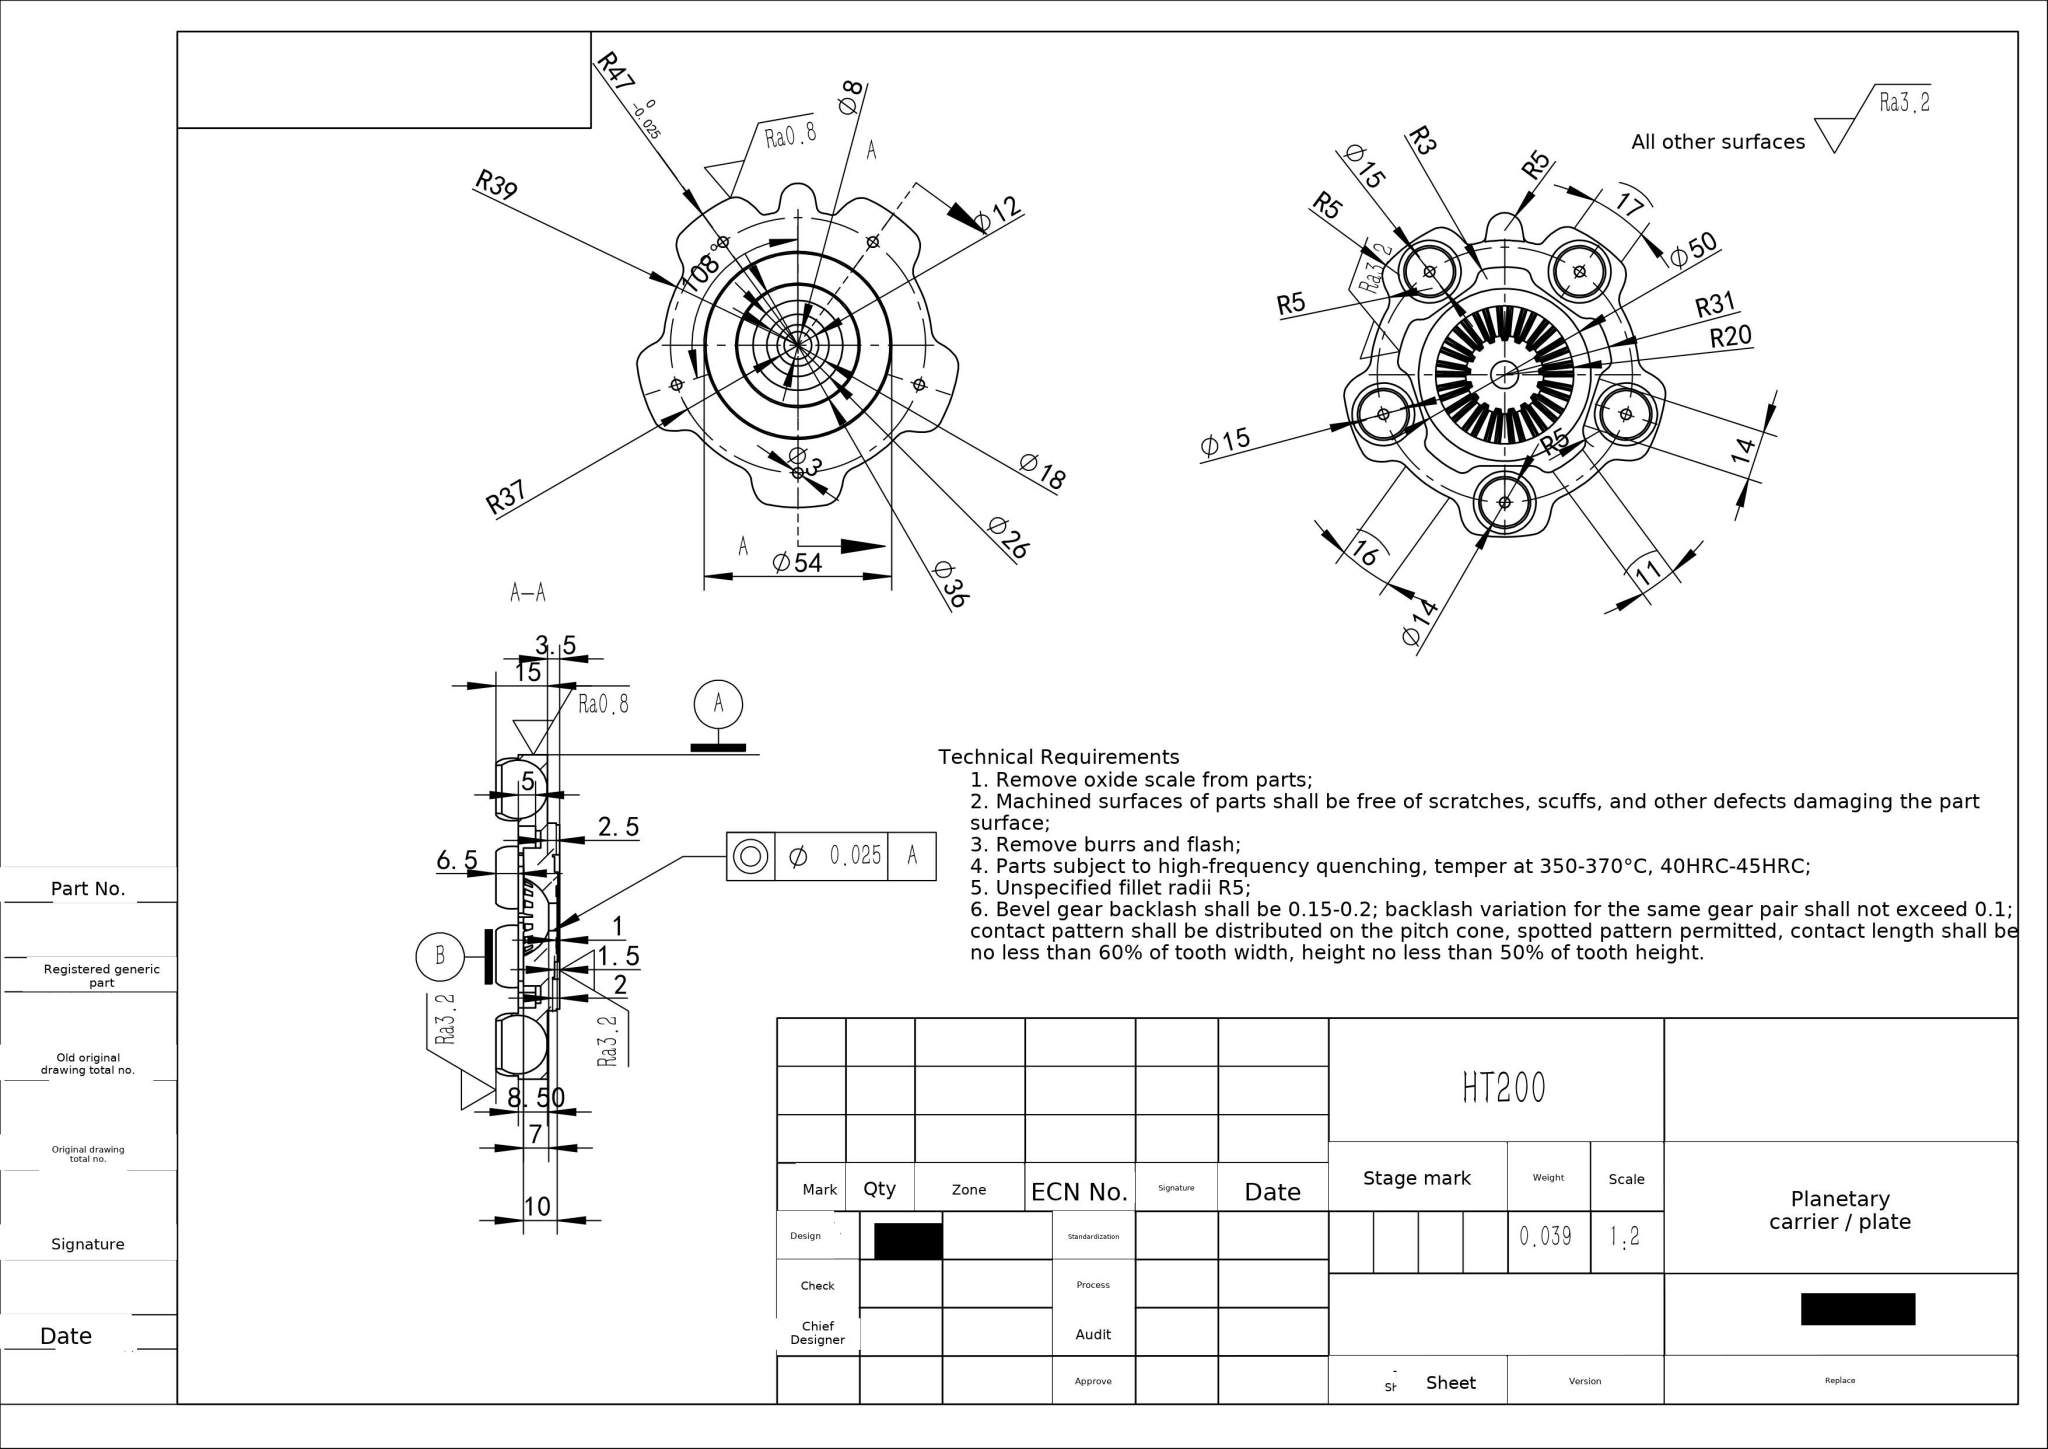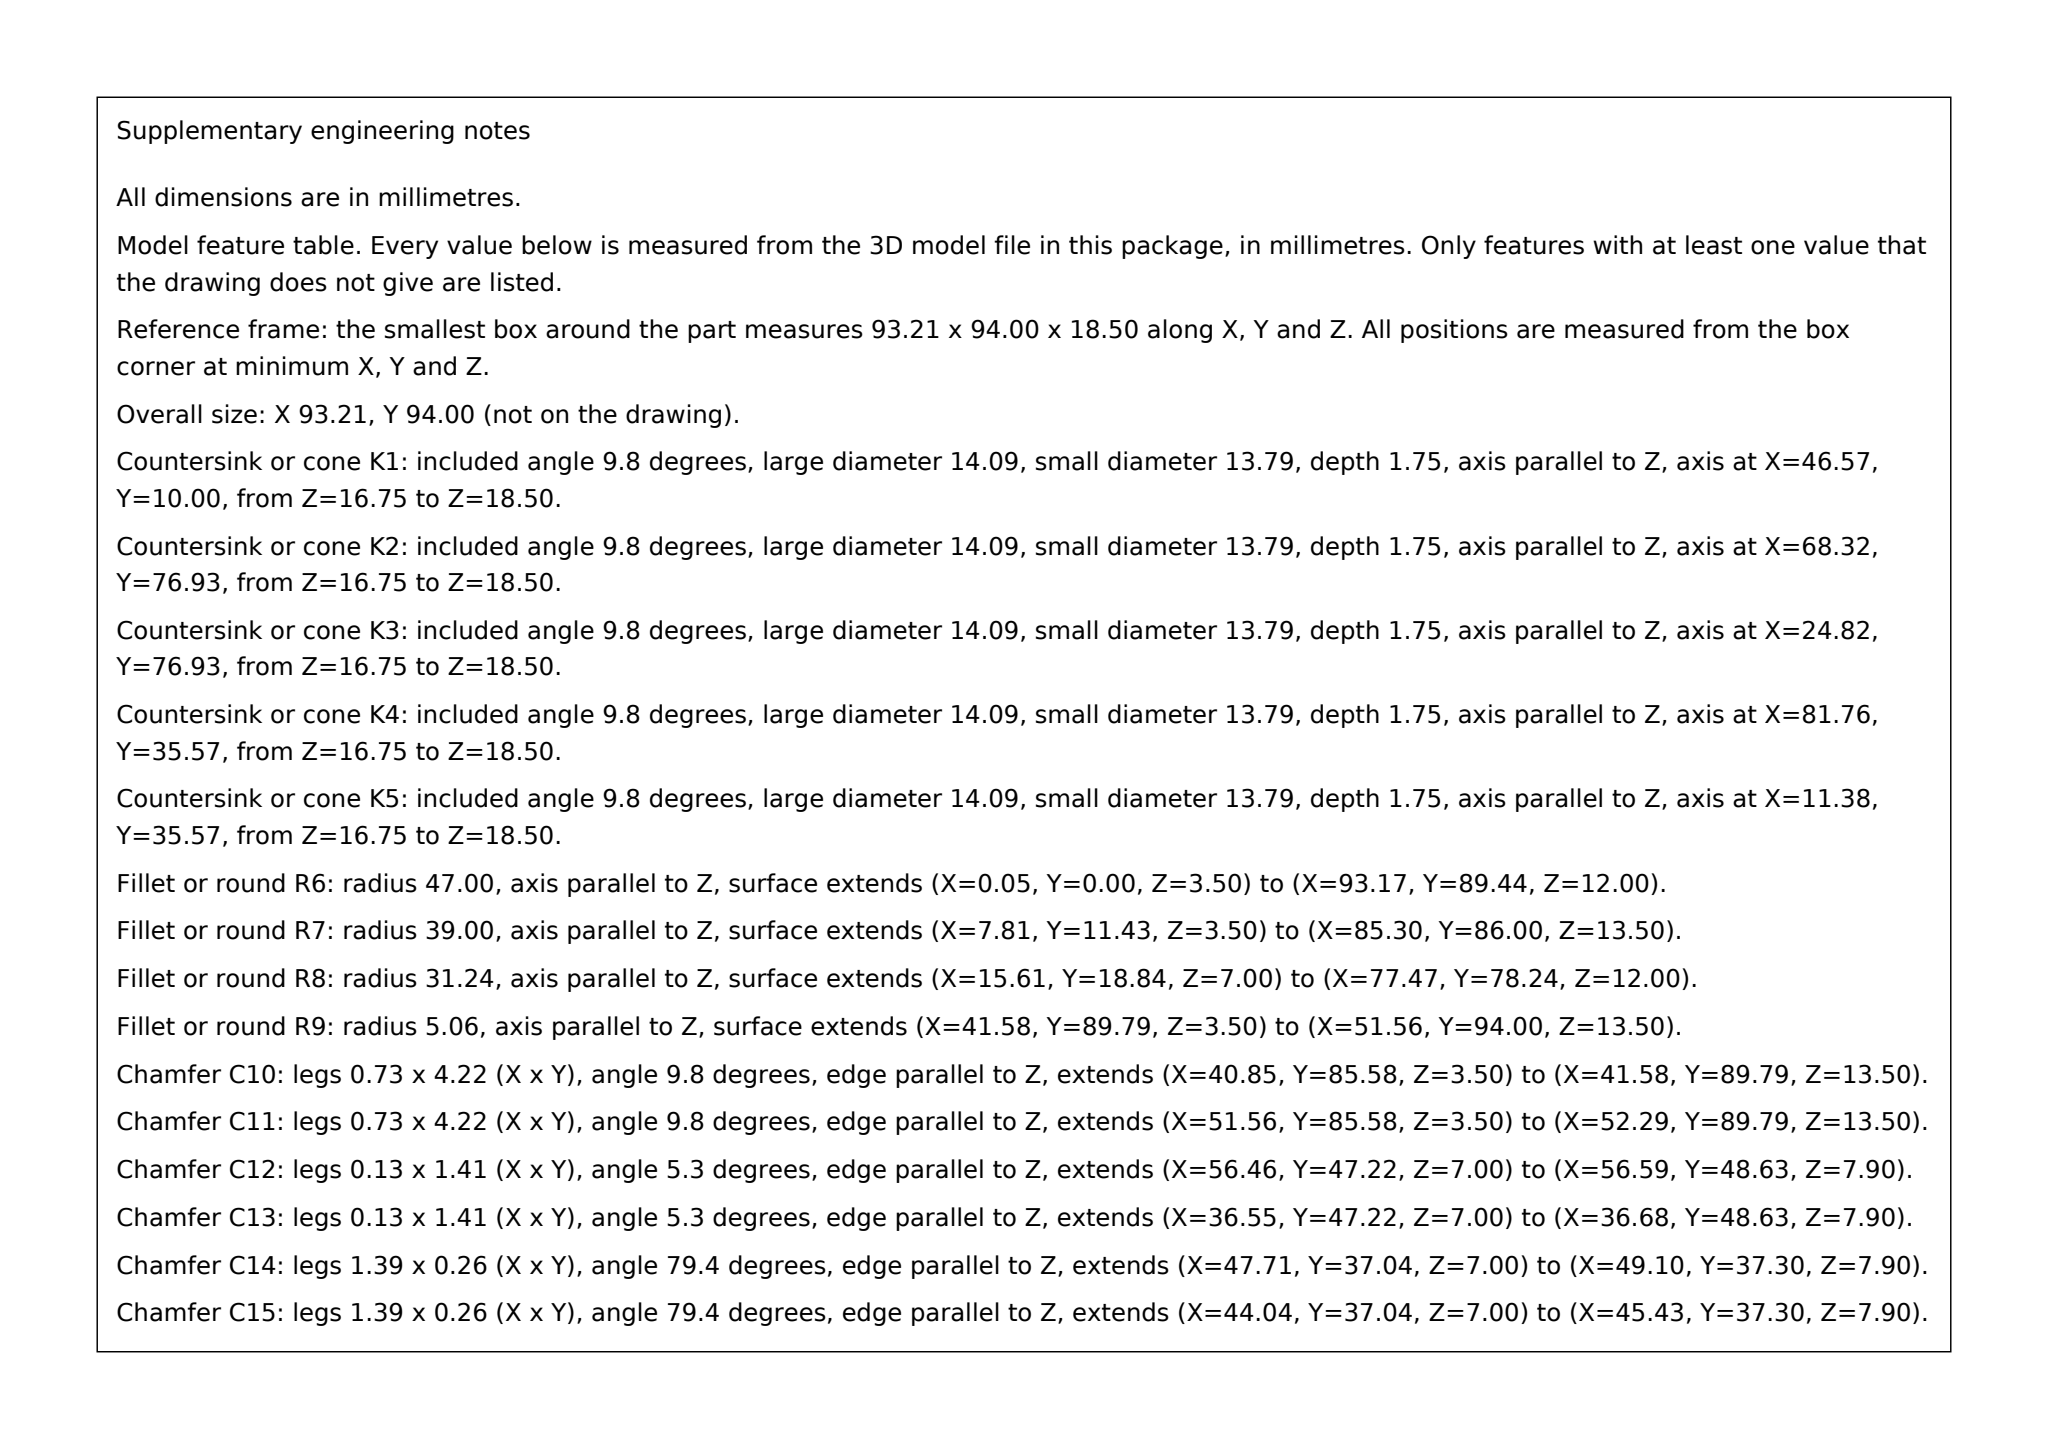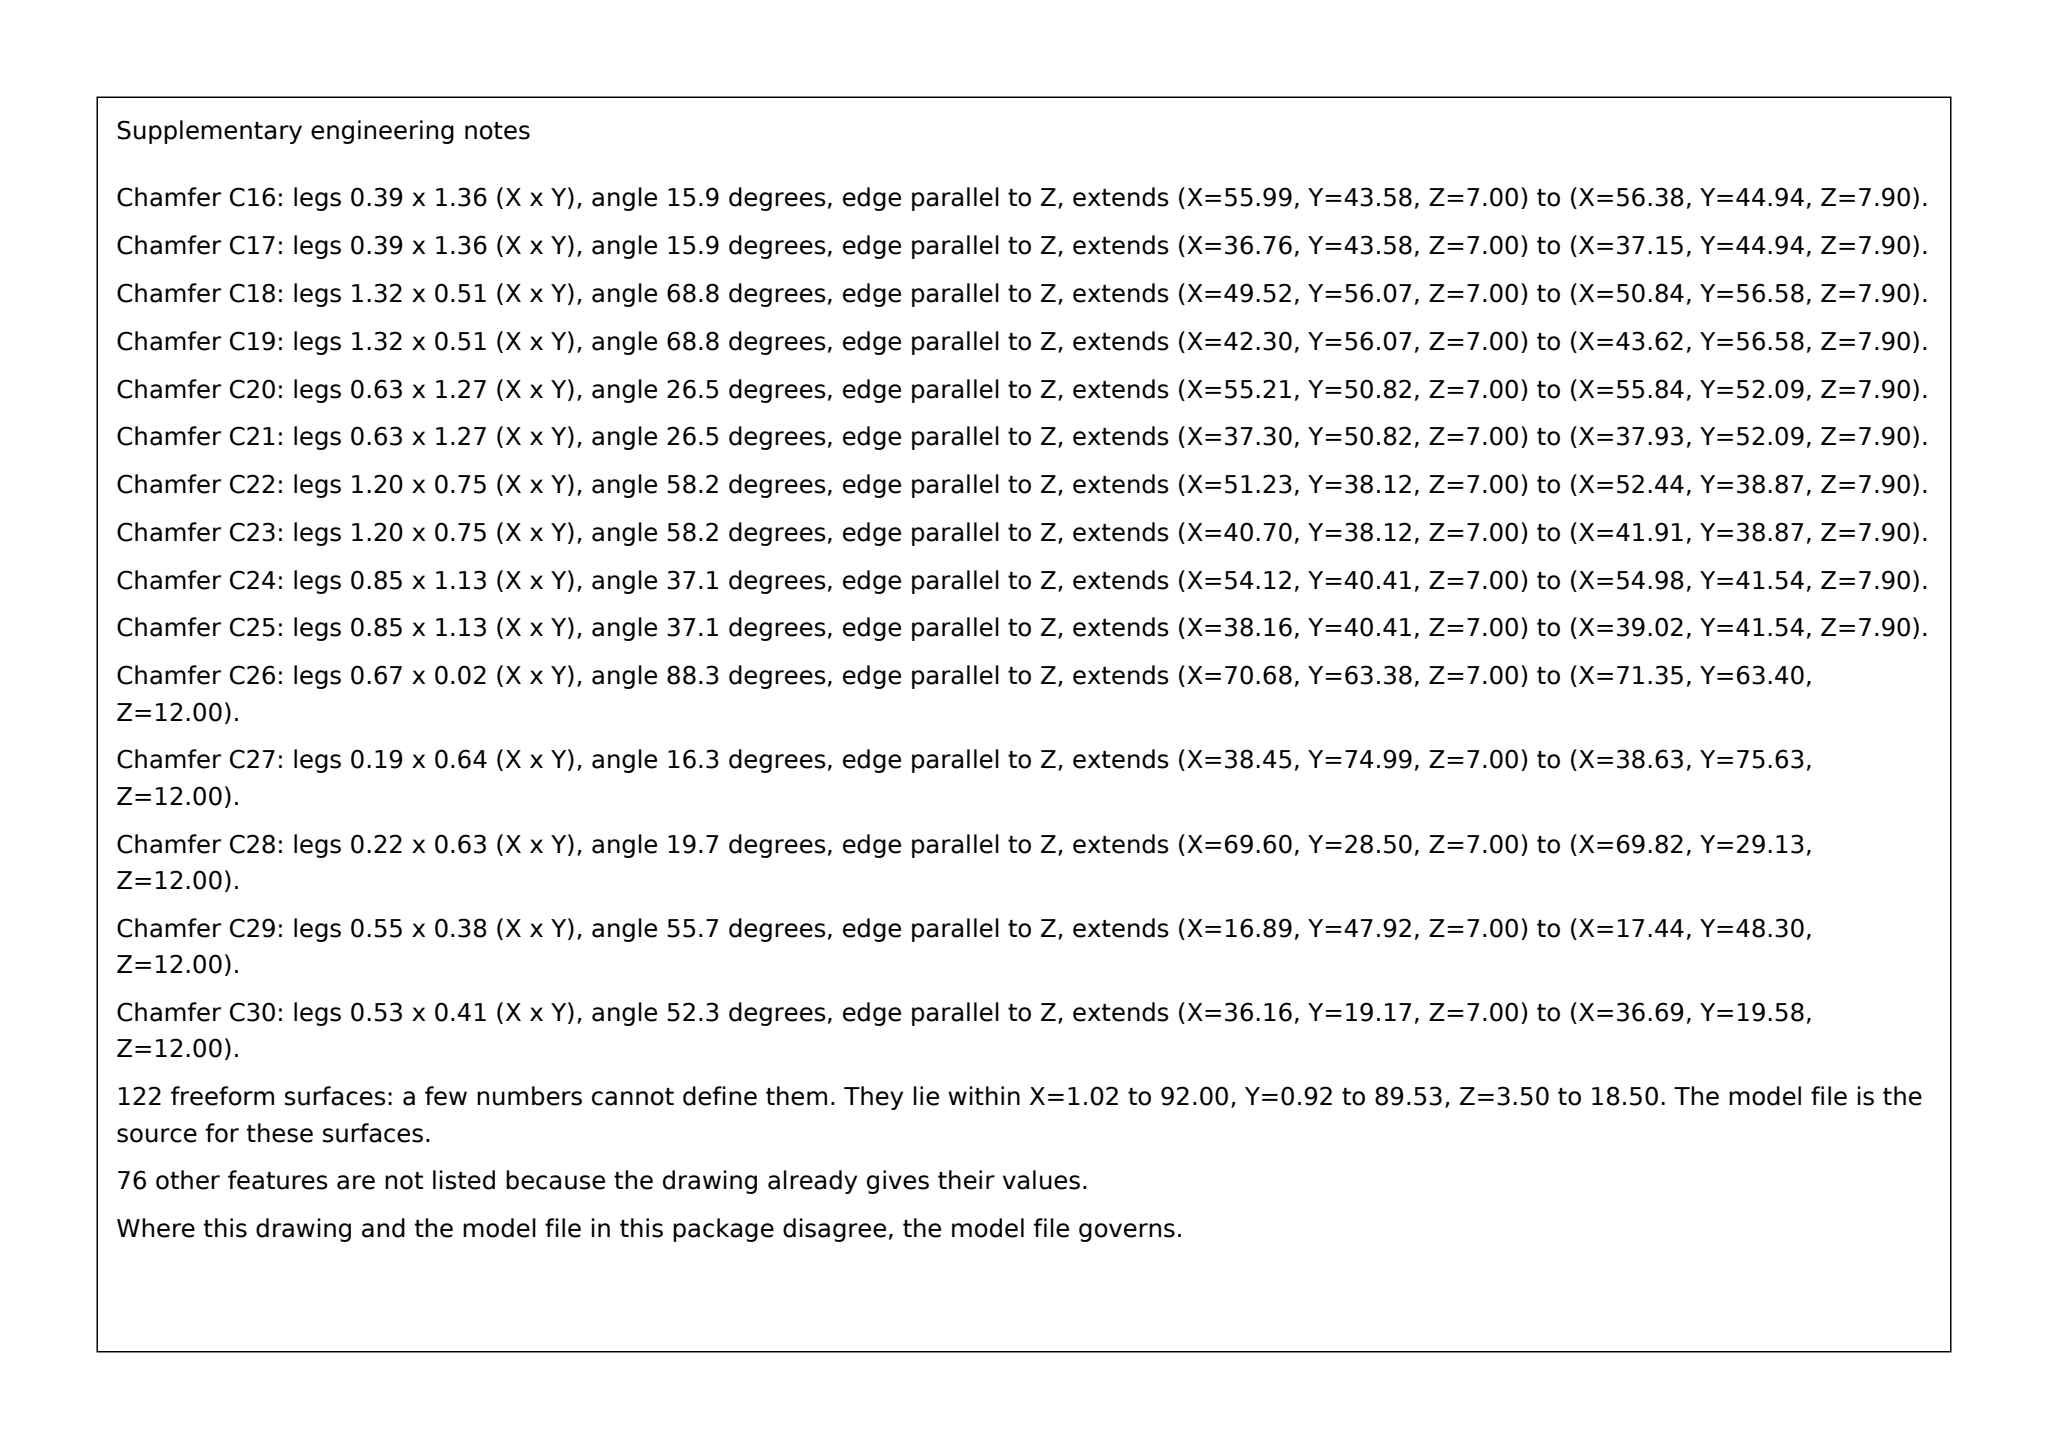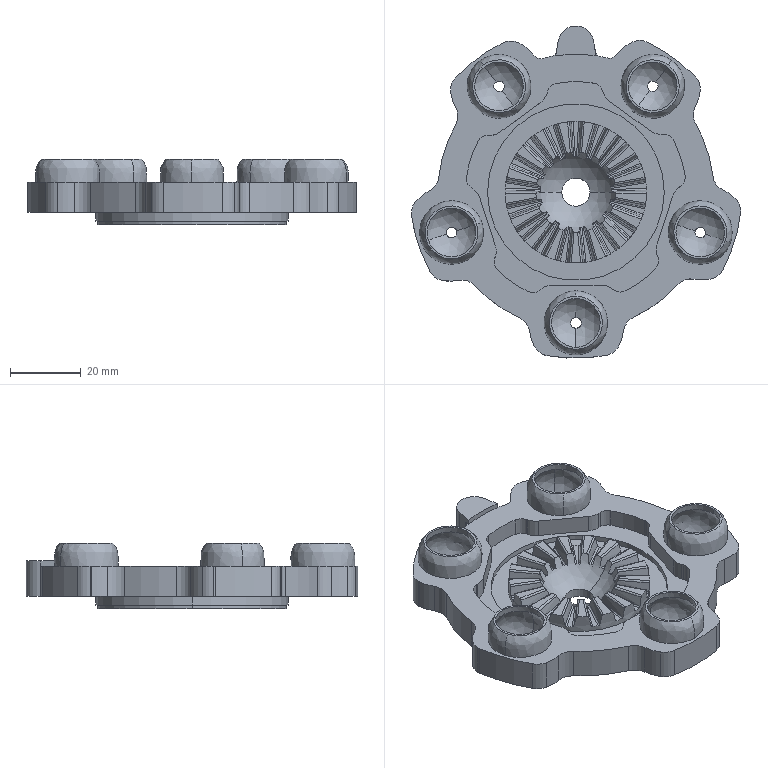Part | SolidWorks | mm | material HT200 | 1 solid | 325 faces | box 93.21 x 94 x 18.5 mm | volume 39278 mm3 | spline 122 | cylinder 96 | plane 85 | sphere 12 | cone 10 | commonest cylinder face diameters 10 x32 6 x12 3 x10 78 x7 94 x5 62.487 x5 4 x4 40 x2